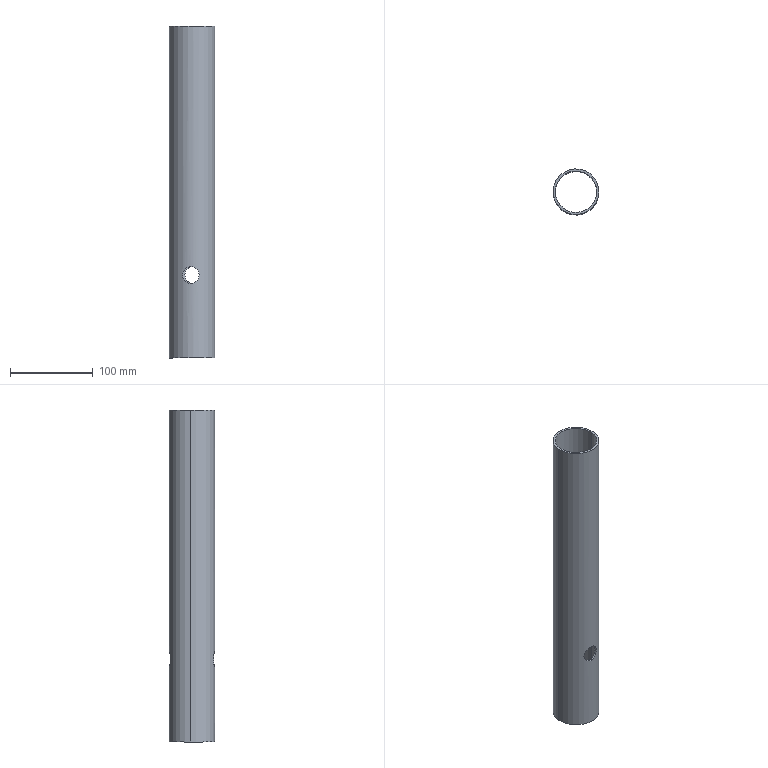Component | SolidWorks | 7LegTravel-2 | 1 solid | 10 faces | box 55 x 55 x 400 mm | volume 163332 mm3 | cylinder 8 | plane 2 | commonest cylinder face diameters 20 x4 50 x2 55 x2
build123d program:
from build123d import *

# Parameters (mm, degrees)
SKETCH1_R           = 27.5
SKETCH1_R_2         = 25
BOSS_EXTRUDE1_DEPTH = 400
SKETCH2_R           = 10
CUT_EXTRUDE1_DEPTH  = 240


with BuildPart() as part:
    # Sketch1 → Boss-Extrude1 (new body)
    with BuildSketch(Plane.XY):
        Circle(SKETCH1_R)
        Circle(SKETCH1_R_2, mode=Mode.SUBTRACT)
    extrude(amount=BOSS_EXTRUDE1_DEPTH)

    # Sketch2 → Cut-Extrude1 (cut, symmetric)
    with BuildSketch(Plane(origin=(0, 25, 0), x_dir=(1, 0, 0), z_dir=(0, 1, 0))):
        with Locations(Location((0, -300, 0), (0, 0, 270))):
            Circle(SKETCH2_R)
    extrude(amount=CUT_EXTRUDE1_DEPTH, both=True, mode=Mode.SUBTRACT)


solid = part.part

# Placed as in the assembly
solid = solid.moved(Location((142.5, 813.71, 917.68), (-180, 0, -176.706)))
STEP:
#1=CARTESIAN_POINT('',(5.548,30.955,24.712));
#2=VERTEX_POINT('',#1);
#3=CARTESIAN_POINT('',(5.548,30.955,23.924));
#4=VERTEX_POINT('',#3);
#5=CARTESIAN_POINT('',(5.548,30.955,24.712));
#6=CARTESIAN_POINT('',(5.561,30.954,24.712));
#7=CARTESIAN_POINT('',(5.574,30.954,24.711));
#8=CARTESIAN_POINT('',(5.6,30.953,24.709));
#9=CARTESIAN_POINT('',(5.613,30.953,24.707));
#10=CARTESIAN_POINT('',(5.651,30.954,24.699));
#11=CARTESIAN_POINT('',(5.676,30.955,24.691));
#12=CARTESIAN_POINT('',(5.712,30.958,24.677));
#13=CARTESIAN_POINT('',(5.724,30.959,24.671));
#14=CARTESIAN_POINT('',(5.747,30.962,24.659));
#15=CARTESIAN_POINT('',(5.758,30.963,24.652));
#16=CARTESIAN_POINT('',(5.79,30.968,24.631));
#17=CARTESIAN_POINT('',(5.81,30.972,24.615));
#18=CARTESIAN_POINT('',(5.847,30.979,24.578));
#19=CARTESIAN_POINT('',(5.863,30.983,24.558));
#20=CARTESIAN_POINT('',(5.885,30.988,24.527));
#21=CARTESIAN_POINT('',(5.891,30.99,24.516));
#22=CARTESIAN_POINT('',(5.904,30.994,24.493));
#23=CARTESIAN_POINT('',(5.91,30.995,24.481));
#24=CARTESIAN_POINT('',(5.925,31.,24.445));
#25=CARTESIAN_POINT('',(5.932,31.002,24.421));
#26=CARTESIAN_POINT('',(5.94,31.005,24.383));
#27=CARTESIAN_POINT('',(5.942,31.005,24.37));
#28=CARTESIAN_POINT('',(5.945,31.006,24.344));
#29=CARTESIAN_POINT('',(5.945,31.006,24.331));
#30=CARTESIAN_POINT('',(5.945,31.006,24.292));
#31=CARTESIAN_POINT('',(5.943,31.005,24.266));
#32=CARTESIAN_POINT('',(5.935,31.003,24.228));
#33=CARTESIAN_POINT('',(5.932,31.002,24.215));
#34=CARTESIAN_POINT('',(5.924,31.,24.191));
#35=CARTESIAN_POINT('',(5.919,30.998,24.178));
#36=CARTESIAN_POINT('',(5.909,30.995,24.155));
#37=CARTESIAN_POINT('',(5.904,30.994,24.143));
#38=CARTESIAN_POINT('',(5.891,30.99,24.12));
#39=CARTESIAN_POINT('',(5.885,30.988,24.109));
#40=CARTESIAN_POINT('',(5.863,30.983,24.077));
#41=CARTESIAN_POINT('',(5.846,30.979,24.058));
#42=CARTESIAN_POINT('',(5.81,30.972,24.022));
#43=CARTESIAN_POINT('',(5.789,30.968,24.005));
#44=CARTESIAN_POINT('',(5.747,30.962,23.977));
#45=CARTESIAN_POINT('',(5.724,30.959,23.965));
#46=CARTESIAN_POINT('',(5.688,30.956,23.95));
#47=CARTESIAN_POINT('',(5.675,30.955,23.945));
#48=CARTESIAN_POINT('',(5.651,30.954,23.938));
#49=CARTESIAN_POINT('',(5.638,30.953,23.935));
#50=CARTESIAN_POINT('',(5.6,30.953,23.927));
#51=CARTESIAN_POINT('',(5.574,30.953,23.924));
#52=CARTESIAN_POINT('',(5.548,30.955,23.924));
#53=B_SPLINE_CURVE_WITH_KNOTS('',3,(#5,#6,#7,#8,#9,#10,#11,#12,#13,#14,#15,#16,#17,#18,#19,#20,#21,#22,#23,#24,#25,#26,#27,#28,#29,#30,#31,#32,#33,#34,#35,#36,#37,#38,#39,#40,#41,#42,#43,#44,#45,#46,#47,#48,#49,#50,#51,#52),.UNSPECIFIED.,.F.,.F.,(4,2,2,2,2,2,2,2,2,2,2,2,2,2,2,2,2,2,2,2,2,2,2,4),(0.03154,0.03252,0.03351,0.03548,0.03646,0.03745,0.03942,0.04139,0.04238,0.04336,0.04533,0.04632,0.0473,0.04927,0.05026,0.05124,0.05223,0.05321,0.05519,0.05716,0.05913,0.06011,0.0611,0.06307),.UNSPECIFIED.);
#54=EDGE_CURVE('',#2,#4,#53,.T.);
#55=ORIENTED_EDGE('',*,*,#54,.F.);
#56=CARTESIAN_POINT('',(5.554,31.053,24.712));
#57=VERTEX_POINT('',#56);
#58=CARTESIAN_POINT('',(5.124,23.585,24.712));
#59=DIRECTION('',(0.05742,0.9983,0.));
#60=VECTOR('',#59,39.37);
#61=LINE('',#58,#60);
#62=EDGE_CURVE('',#2,#57,#61,.T.);
#63=ORIENTED_EDGE('',*,*,#62,.T.);
#64=CARTESIAN_POINT('',(5.554,31.053,23.924));
#65=VERTEX_POINT('',#64);
#66=CARTESIAN_POINT('',(5.554,31.053,24.712));
#67=CARTESIAN_POINT('',(5.567,31.052,24.712));
#68=CARTESIAN_POINT('',(5.58,31.052,24.711));
#69=CARTESIAN_POINT('',(5.606,31.051,24.709));
#70=CARTESIAN_POINT('',(5.619,31.052,24.707));
#71=CARTESIAN_POINT('',(5.657,31.052,24.699));
#72=CARTESIAN_POINT('',(5.682,31.054,24.691));
#73=CARTESIAN_POINT('',(5.718,31.057,24.676));
#74=CARTESIAN_POINT('',(5.73,31.059,24.671));
#75=CARTESIAN_POINT('',(5.753,31.062,24.659));
#76=CARTESIAN_POINT('',(5.764,31.064,24.652));
#77=CARTESIAN_POINT('',(5.796,31.069,24.631));
#78=CARTESIAN_POINT('',(5.816,31.073,24.614));
#79=CARTESIAN_POINT('',(5.853,31.082,24.578));
#80=CARTESIAN_POINT('',(5.869,31.086,24.558));
#81=CARTESIAN_POINT('',(5.891,31.092,24.527));
#82=CARTESIAN_POINT('',(5.897,31.094,24.516));
#83=CARTESIAN_POINT('',(5.91,31.098,24.493));
#84=CARTESIAN_POINT('',(5.915,31.1,24.481));
#85=CARTESIAN_POINT('',(5.931,31.105,24.446));
#86=CARTESIAN_POINT('',(5.938,31.108,24.421));
#87=CARTESIAN_POINT('',(5.946,31.111,24.383));
#88=CARTESIAN_POINT('',(5.948,31.111,24.37));
#89=CARTESIAN_POINT('',(5.951,31.112,24.344));
#90=CARTESIAN_POINT('',(5.951,31.113,24.331));
#91=CARTESIAN_POINT('',(5.951,31.113,24.292));
#92=CARTESIAN_POINT('',(5.949,31.112,24.266));
#93=CARTESIAN_POINT('',(5.941,31.109,24.228));
#94=CARTESIAN_POINT('',(5.938,31.108,24.215));
#95=CARTESIAN_POINT('',(5.93,31.105,24.191));
#96=CARTESIAN_POINT('',(5.926,31.103,24.178));
#97=CARTESIAN_POINT('',(5.915,31.1,24.155));
#98=CARTESIAN_POINT('',(5.91,31.098,24.143));
#99=CARTESIAN_POINT('',(5.897,31.094,24.12));
#100=CARTESIAN_POINT('',(5.891,31.092,24.109));
#101=CARTESIAN_POINT('',(5.869,31.086,24.078));
#102=CARTESIAN_POINT('',(5.852,31.082,24.058));
#103=CARTESIAN_POINT('',(5.825,31.075,24.031));
#104=CARTESIAN_POINT('',(5.815,31.073,24.022));
#105=CARTESIAN_POINT('',(5.795,31.069,24.006));
#106=CARTESIAN_POINT('',(5.785,31.067,23.998));
#107=CARTESIAN_POINT('',(5.753,31.062,23.977));
#108=CARTESIAN_POINT('',(5.73,31.059,23.965));
#109=CARTESIAN_POINT('',(5.694,31.055,23.95));
#110=CARTESIAN_POINT('',(5.681,31.054,23.945));
#111=CARTESIAN_POINT('',(5.657,31.053,23.938));
#112=CARTESIAN_POINT('',(5.644,31.052,23.935));
#113=CARTESIAN_POINT('',(5.619,31.052,23.93));
#114=CARTESIAN_POINT('',(5.606,31.051,23.928));
#115=CARTESIAN_POINT('',(5.58,31.052,23.925));
#116=CARTESIAN_POINT('',(5.567,31.052,23.924));
#117=CARTESIAN_POINT('',(5.554,31.053,23.924));
#118=B_SPLINE_CURVE_WITH_KNOTS('',3,(#66,#67,#68,#69,#70,#71,#72,#73,#74,#75,#76,#77,#78,#79,#80,#81,#82,#83,#84,#85,#86,#87,#88,#89,#90,#91,#92,#93,#94,#95,#96,#97,#98,#99,#100,#101,#102,#103,#104,#105,#106,#107,#108,#109,#110,#111,#112,#113,#114,#115,#116,#117),.UNSPECIFIED.,.F.,.F.,(4,2,2,2,2,2,2,2,2,2,2,2,2,2,2,2,2,2,2,2,2,2,2,2,2,4),(0.0316,0.03259,0.03357,0.03555,0.03653,0.03752,0.03949,0.04147,0.04245,0.04344,0.04541,0.0464,0.04739,0.04936,0.05035,0.05134,0.05232,0.05331,0.05528,0.05627,0.05726,0.05923,0.06022,0.0612,0.06219,0.06318),.UNSPECIFIED.);
#119=EDGE_CURVE('',#57,#65,#118,.T.);
#120=ORIENTED_EDGE('',*,*,#119,.T.);
#121=CARTESIAN_POINT('',(5.124,23.585,23.924));
#122=DIRECTION('',(0.05742,0.9983,0.));
#123=VECTOR('',#122,39.37);
#124=LINE('',#121,#123);
#125=EDGE_CURVE('',#4,#65,#124,.T.);
#126=ORIENTED_EDGE('',*,*,#125,.F.);
#127=EDGE_LOOP('',(#55,#63,#120,#126));
#128=FACE_OUTER_BOUND('',#127,.T.);
#129=CARTESIAN_POINT('',(5.124,23.585,24.318));
#130=DIRECTION('',(0.05742,0.9983,0.));
#131=DIRECTION('',(0.,0.,-1.));
#132=AXIS2_PLACEMENT_3D('',#129,#130,#131);
#133=CYLINDRICAL_SURFACE('',#132,0.3937);
#134=ADVANCED_FACE('',(#128),#133,.F.);
#135=CARTESIAN_POINT('',(5.667,33.018,23.924));
#136=VERTEX_POINT('',#135);
#137=CARTESIAN_POINT('',(5.667,33.018,24.712));
#138=VERTEX_POINT('',#137);
#139=CARTESIAN_POINT('',(5.667,33.018,23.924));
#140=CARTESIAN_POINT('',(5.693,33.017,23.924));
#141=CARTESIAN_POINT('',(5.719,33.014,23.927));
#142=CARTESIAN_POINT('',(5.757,33.009,23.935));
#143=CARTESIAN_POINT('',(5.769,33.007,23.938));
#144=CARTESIAN_POINT('',(5.794,33.003,23.945));
#145=CARTESIAN_POINT('',(5.806,33.001,23.95));
#146=CARTESIAN_POINT('',(5.841,32.993,23.965));
#147=CARTESIAN_POINT('',(5.863,32.987,23.977));
#148=CARTESIAN_POINT('',(5.895,32.978,23.998));
#149=CARTESIAN_POINT('',(5.905,32.975,24.006));
#150=CARTESIAN_POINT('',(5.924,32.969,24.022));
#151=CARTESIAN_POINT('',(5.934,32.965,24.031));
#152=CARTESIAN_POINT('',(5.96,32.956,24.058));
#153=CARTESIAN_POINT('',(5.976,32.95,24.078));
#154=CARTESIAN_POINT('',(6.004,32.938,24.12));
#155=CARTESIAN_POINT('',(6.016,32.933,24.143));
#156=CARTESIAN_POINT('',(6.03,32.926,24.178));
#157=CARTESIAN_POINT('',(6.035,32.924,24.19));
#158=CARTESIAN_POINT('',(6.042,32.92,24.215));
#159=CARTESIAN_POINT('',(6.045,32.919,24.228));
#160=CARTESIAN_POINT('',(6.053,32.915,24.266));
#161=CARTESIAN_POINT('',(6.055,32.914,24.292));
#162=CARTESIAN_POINT('',(6.055,32.914,24.331));
#163=CARTESIAN_POINT('',(6.054,32.914,24.344));
#164=CARTESIAN_POINT('',(6.052,32.915,24.37));
#165=CARTESIAN_POINT('',(6.05,32.916,24.383));
#166=CARTESIAN_POINT('',(6.043,32.92,24.421));
#167=CARTESIAN_POINT('',(6.035,32.924,24.446));
#168=CARTESIAN_POINT('',(6.016,32.933,24.494));
#169=CARTESIAN_POINT('',(6.004,32.938,24.516));
#170=CARTESIAN_POINT('',(5.983,32.947,24.548));
#171=CARTESIAN_POINT('',(5.976,32.95,24.558));
#172=CARTESIAN_POINT('',(5.96,32.956,24.578));
#173=CARTESIAN_POINT('',(5.951,32.959,24.588));
#174=CARTESIAN_POINT('',(5.925,32.969,24.615));
#175=CARTESIAN_POINT('',(5.905,32.975,24.631));
#176=CARTESIAN_POINT('',(5.874,32.984,24.652));
#177=CARTESIAN_POINT('',(5.863,32.987,24.659));
#178=CARTESIAN_POINT('',(5.84,32.993,24.671));
#179=CARTESIAN_POINT('',(5.829,32.996,24.677));
#180=CARTESIAN_POINT('',(5.794,33.003,24.691));
#181=CARTESIAN_POINT('',(5.769,33.007,24.699));
#182=CARTESIAN_POINT('',(5.731,33.013,24.707));
#183=CARTESIAN_POINT('',(5.718,33.014,24.709));
#184=CARTESIAN_POINT('',(5.693,33.017,24.711));
#185=CARTESIAN_POINT('',(5.68,33.018,24.712));
#186=CARTESIAN_POINT('',(5.667,33.018,24.712));
#187=B_SPLINE_CURVE_WITH_KNOTS('',3,(#139,#140,#141,#142,#143,#144,#145,#146,#147,#148,#149,#150,#151,#152,#153,#154,#155,#156,#157,#158,#159,#160,#161,#162,#163,#164,#165,#166,#167,#168,#169,#170,#171,#172,#173,#174,#175,#176,#177,#178,#179,#180,#181,#182,#183,#184,#185,#186),.UNSPECIFIED.,.F.,.F.,(4,2,2,2,2,2,2,2,2,2,2,2,2,2,2,2,2,2,2,2,2,2,2,4),(0.,0.001975,0.002962,0.00395,0.005925,0.006912,0.0079,0.009875,0.01185,0.01284,0.01382,0.0158,0.01679,0.01777,0.01975,0.02172,0.02271,0.0237,0.02567,0.02666,0.02765,0.02962,0.03061,0.0316),.UNSPECIFIED.);
#188=EDGE_CURVE('',#136,#138,#187,.T.);
#189=ORIENTED_EDGE('',*,*,#188,.T.);
#190=CARTESIAN_POINT('',(5.672,33.117,24.712));
#191=VERTEX_POINT('',#190);
#192=CARTESIAN_POINT('',(5.124,23.585,24.712));
#193=DIRECTION('',(0.05742,0.9983,0.));
#194=VECTOR('',#193,39.37);
#195=LINE('',#192,#194);
#196=EDGE_CURVE('',#138,#191,#195,.T.);
#197=ORIENTED_EDGE('',*,*,#196,.T.);
#198=CARTESIAN_POINT('',(5.672,33.117,23.924));
#199=VERTEX_POINT('',#198);
#200=CARTESIAN_POINT('',(5.672,33.117,23.924));
#201=CARTESIAN_POINT('',(5.699,33.115,23.924));
#202=CARTESIAN_POINT('',(5.724,33.113,23.927));
#203=CARTESIAN_POINT('',(5.762,33.108,23.935));
#204=CARTESIAN_POINT('',(5.774,33.106,23.938));
#205=CARTESIAN_POINT('',(5.799,33.102,23.945));
#206=CARTESIAN_POINT('',(5.811,33.1,23.95));
#207=CARTESIAN_POINT('',(5.847,33.093,23.965));
#208=CARTESIAN_POINT('',(5.869,33.087,23.977));
#209=CARTESIAN_POINT('',(5.9,33.079,23.998));
#210=CARTESIAN_POINT('',(5.911,33.076,24.006));
#211=CARTESIAN_POINT('',(5.93,33.07,24.022));
#212=CARTESIAN_POINT('',(5.94,33.067,24.031));
#213=CARTESIAN_POINT('',(5.966,33.059,24.058));
#214=CARTESIAN_POINT('',(5.982,33.053,24.078));
#215=CARTESIAN_POINT('',(6.01,33.042,24.12));
#216=CARTESIAN_POINT('',(6.022,33.037,24.143));
#217=CARTESIAN_POINT('',(6.036,33.031,24.178));
#218=CARTESIAN_POINT('',(6.041,33.029,24.191));
#219=CARTESIAN_POINT('',(6.048,33.026,24.215));
#220=CARTESIAN_POINT('',(6.051,33.025,24.228));
#221=CARTESIAN_POINT('',(6.059,33.021,24.266));
#222=CARTESIAN_POINT('',(6.061,33.02,24.292));
#223=CARTESIAN_POINT('',(6.061,33.02,24.331));
#224=CARTESIAN_POINT('',(6.061,33.02,24.344));
#225=CARTESIAN_POINT('',(6.058,33.022,24.37));
#226=CARTESIAN_POINT('',(6.056,33.022,24.383));
#227=CARTESIAN_POINT('',(6.049,33.026,24.421));
#228=CARTESIAN_POINT('',(6.041,33.029,24.446));
#229=CARTESIAN_POINT('',(6.022,33.037,24.493));
#230=CARTESIAN_POINT('',(6.01,33.042,24.516));
#231=CARTESIAN_POINT('',(5.989,33.05,24.548));
#232=CARTESIAN_POINT('',(5.982,33.053,24.558));
#233=CARTESIAN_POINT('',(5.966,33.059,24.578));
#234=CARTESIAN_POINT('',(5.957,33.061,24.588));
#235=CARTESIAN_POINT('',(5.93,33.07,24.615));
#236=CARTESIAN_POINT('',(5.911,33.076,24.631));
#237=CARTESIAN_POINT('',(5.88,33.085,24.652));
#238=CARTESIAN_POINT('',(5.869,33.087,24.659));
#239=CARTESIAN_POINT('',(5.846,33.093,24.671));
#240=CARTESIAN_POINT('',(5.835,33.095,24.677));
#241=CARTESIAN_POINT('',(5.799,33.102,24.691));
#242=CARTESIAN_POINT('',(5.775,33.106,24.699));
#243=CARTESIAN_POINT('',(5.737,33.111,24.707));
#244=CARTESIAN_POINT('',(5.724,33.113,24.709));
#245=CARTESIAN_POINT('',(5.698,33.115,24.711));
#246=CARTESIAN_POINT('',(5.685,33.116,24.712));
#247=CARTESIAN_POINT('',(5.672,33.117,24.712));
#248=B_SPLINE_CURVE_WITH_KNOTS('',3,(#200,#201,#202,#203,#204,#205,#206,#207,#208,#209,#210,#211,#212,#213,#214,#215,#216,#217,#218,#219,#220,#221,#222,#223,#224,#225,#226,#227,#228,#229,#230,#231,#232,#233,#234,#235,#236,#237,#238,#239,#240,#241,#242,#243,#244,#245,#246,#247),.UNSPECIFIED.,.F.,.F.,(4,2,2,2,2,2,2,2,2,2,2,2,2,2,2,2,2,2,2,2,2,2,2,4),(0.,0.001971,0.002957,0.003942,0.005913,0.006899,0.007884,0.009855,0.01183,0.01281,0.0138,0.01577,0.01675,0.01774,0.01971,0.02168,0.02267,0.02365,0.02562,0.02661,0.0276,0.02957,0.03055,0.03154),.UNSPECIFIED.);
#249=EDGE_CURVE('',#199,#191,#248,.T.);
#250=ORIENTED_EDGE('',*,*,#249,.F.);
#251=CARTESIAN_POINT('',(5.124,23.585,23.924));
#252=DIRECTION('',(0.05742,0.9983,0.));
#253=VECTOR('',#252,39.37);
#254=LINE('',#251,#253);
#255=EDGE_CURVE('',#136,#199,#254,.T.);
#256=ORIENTED_EDGE('',*,*,#255,.F.);
#257=EDGE_LOOP('',(#189,#197,#250,#256));
#258=FACE_OUTER_BOUND('',#257,.T.);
#259=CARTESIAN_POINT('',(5.124,23.585,24.318));
#260=DIRECTION('',(0.05742,0.9983,0.));
#261=DIRECTION('',(0.,0.,-1.));
#262=AXIS2_PLACEMENT_3D('',#259,#260,#261);
#263=CYLINDRICAL_SURFACE('',#262,0.3937);
#264=ADVANCED_FACE('',(#258),#263,.F.);
#265=CARTESIAN_POINT('',(5.554,31.053,23.924));
#266=CARTESIAN_POINT('',(5.527,31.055,23.924));
#267=CARTESIAN_POINT('',(5.502,31.057,23.927));
#268=CARTESIAN_POINT('',(5.464,31.062,23.935));
#269=CARTESIAN_POINT('',(5.451,31.064,23.938));
#270=CARTESIAN_POINT('',(5.427,31.069,23.945));
#271=CARTESIAN_POINT('',(5.415,31.071,23.95));
#272=CARTESIAN_POINT('',(5.379,31.079,23.965));
#273=CARTESIAN_POINT('',(5.357,31.084,23.977));
#274=CARTESIAN_POINT('',(5.326,31.094,23.998));
#275=CARTESIAN_POINT('',(5.315,31.097,24.006));
#276=CARTESIAN_POINT('',(5.296,31.103,24.022));
#277=CARTESIAN_POINT('',(5.287,31.106,24.031));
#278=CARTESIAN_POINT('',(5.26,31.116,24.058));
#279=CARTESIAN_POINT('',(5.244,31.122,24.078));
#280=CARTESIAN_POINT('',(5.216,31.134,24.12));
#281=CARTESIAN_POINT('',(5.205,31.139,24.143));
#282=CARTESIAN_POINT('',(5.19,31.146,24.178));
#283=CARTESIAN_POINT('',(5.186,31.148,24.19));
#284=CARTESIAN_POINT('',(5.178,31.151,24.215));
#285=CARTESIAN_POINT('',(5.175,31.153,24.228));
#286=CARTESIAN_POINT('',(5.168,31.157,24.266));
#287=CARTESIAN_POINT('',(5.165,31.158,24.292));
#288=CARTESIAN_POINT('',(5.165,31.158,24.331));
#289=CARTESIAN_POINT('',(5.166,31.158,24.344));
#290=CARTESIAN_POINT('',(5.169,31.156,24.37));
#291=CARTESIAN_POINT('',(5.17,31.155,24.383));
#292=CARTESIAN_POINT('',(5.178,31.152,24.421));
#293=CARTESIAN_POINT('',(5.185,31.148,24.446));
#294=CARTESIAN_POINT('',(5.205,31.139,24.494));
#295=CARTESIAN_POINT('',(5.217,31.134,24.516));
#296=CARTESIAN_POINT('',(5.237,31.125,24.548));
#297=CARTESIAN_POINT('',(5.245,31.122,24.558));
#298=CARTESIAN_POINT('',(5.261,31.116,24.578));
#299=CARTESIAN_POINT('',(5.269,31.112,24.588));
#300=CARTESIAN_POINT('',(5.296,31.103,24.615));
#301=CARTESIAN_POINT('',(5.315,31.097,24.631));
#302=CARTESIAN_POINT('',(5.347,31.087,24.652));
#303=CARTESIAN_POINT('',(5.358,31.084,24.659));
#304=CARTESIAN_POINT('',(5.38,31.079,24.671));
#305=CARTESIAN_POINT('',(5.391,31.076,24.677));
#306=CARTESIAN_POINT('',(5.427,31.069,24.691));
#307=CARTESIAN_POINT('',(5.451,31.064,24.699));
#308=CARTESIAN_POINT('',(5.489,31.059,24.707));
#309=CARTESIAN_POINT('',(5.502,31.057,24.709));
#310=CARTESIAN_POINT('',(5.528,31.055,24.711));
#311=CARTESIAN_POINT('',(5.541,31.054,24.712));
#312=CARTESIAN_POINT('',(5.554,31.053,24.712));
#313=B_SPLINE_CURVE_WITH_KNOTS('',3,(#265,#266,#267,#268,#269,#270,#271,#272,#273,#274,#275,#276,#277,#278,#279,#280,#281,#282,#283,#284,#285,#286,#287,#288,#289,#290,#291,#292,#293,#294,#295,#296,#297,#298,#299,#300,#301,#302,#303,#304,#305,#306,#307,#308,#309,#310,#311,#312),.UNSPECIFIED.,.F.,.F.,(4,2,2,2,2,2,2,2,2,2,2,2,2,2,2,2,2,2,2,2,2,2,2,4),(0.,0.001975,0.002962,0.00395,0.005925,0.006912,0.0079,0.009875,0.01185,0.01284,0.01382,0.0158,0.01679,0.01777,0.01975,0.02172,0.02271,0.0237,0.02567,0.02666,0.02765,0.02962,0.03061,0.0316),.UNSPECIFIED.);
#314=EDGE_CURVE('',#65,#57,#313,.T.);
#315=ORIENTED_EDGE('',*,*,#314,.F.);
#316=ORIENTED_EDGE('',*,*,#119,.F.);
#317=EDGE_LOOP('',(#315,#316));
#318=FACE_BOUND('',#317,.T.);
#319=CARTESIAN_POINT('',(6.593,31.979,20.381));
#320=VERTEX_POINT('',#319);
#321=CARTESIAN_POINT('',(4.628,32.092,20.381));
#322=VERTEX_POINT('',#321);
#323=CARTESIAN_POINT('',(5.61,32.036,20.381));
#324=DIRECTION('',(0.,0.,-1.));
#325=DIRECTION('',(-0.9983,0.05742,-0.));
#326=AXIS2_PLACEMENT_3D('',#323,#324,#325);
#327=CIRCLE('',#326,0.9843);
#328=EDGE_CURVE('',#320,#322,#327,.T.);
#329=ORIENTED_EDGE('',*,*,#328,.T.);
#330=CARTESIAN_POINT('',(4.628,32.092,36.129));
#331=VERTEX_POINT('',#330);
#332=CARTESIAN_POINT('',(4.628,32.092,20.381));
#333=DIRECTION('',(-0.,-0.,1.));
#334=VECTOR('',#333,39.37);
#335=LINE('',#332,#334);
#336=EDGE_CURVE('',#322,#331,#335,.T.);
#337=ORIENTED_EDGE('',*,*,#336,.T.);
#338=CARTESIAN_POINT('',(6.593,31.979,36.129));
#339=VERTEX_POINT('',#338);
#340=CARTESIAN_POINT('',(5.61,32.036,36.129));
#341=DIRECTION('',(0.,0.,-1.));
#342=DIRECTION('',(-0.9983,0.05742,-0.));
#343=AXIS2_PLACEMENT_3D('',#340,#341,#342);
#344=CIRCLE('',#343,0.9843);
#345=EDGE_CURVE('',#339,#331,#344,.T.);
#346=ORIENTED_EDGE('',*,*,#345,.F.);
#347=CARTESIAN_POINT('',(6.593,31.979,20.381));
#348=DIRECTION('',(-0.,-0.,1.));
#349=VECTOR('',#348,39.37);
#350=LINE('',#347,#349);
#351=EDGE_CURVE('',#320,#339,#350,.T.);
#352=ORIENTED_EDGE('',*,*,#351,.F.);
#353=EDGE_LOOP('',(#329,#337,#346,#352));
#354=FACE_OUTER_BOUND('',#353,.T.);
#355=CARTESIAN_POINT('',(5.61,32.036,20.381));
#356=DIRECTION('',(-0.,-0.,1.));
#357=DIRECTION('',(0.9983,-0.05742,0.));
#358=AXIS2_PLACEMENT_3D('',#355,#356,#357);
#359=CYLINDRICAL_SURFACE('',#358,0.9843);
#360=ADVANCED_FACE('',(#318,#354),#359,.F.);
#361=ORIENTED_EDGE('',*,*,#249,.T.);
#362=CARTESIAN_POINT('',(5.672,33.117,24.712));
#363=CARTESIAN_POINT('',(5.659,33.117,24.712));
#364=CARTESIAN_POINT('',(5.647,33.118,24.711));
#365=CARTESIAN_POINT('',(5.621,33.119,24.709));
#366=CARTESIAN_POINT('',(5.608,33.119,24.707));
#367=CARTESIAN_POINT('',(5.569,33.118,24.699));
#368=CARTESIAN_POINT('',(5.545,33.117,24.691));
#369=CARTESIAN_POINT('',(5.509,33.114,24.677));
#370=CARTESIAN_POINT('',(5.497,33.113,24.671));
#371=CARTESIAN_POINT('',(5.474,33.11,24.659));
#372=CARTESIAN_POINT('',(5.463,33.108,24.652));
#373=CARTESIAN_POINT('',(5.431,33.104,24.631));
#374=CARTESIAN_POINT('',(5.411,33.1,24.615));
#375=CARTESIAN_POINT('',(5.374,33.093,24.578));
#376=CARTESIAN_POINT('',(5.357,33.089,24.558));
#377=CARTESIAN_POINT('',(5.336,33.083,24.527));
#378=CARTESIAN_POINT('',(5.329,33.081,24.516));
#379=CARTESIAN_POINT('',(5.317,33.078,24.493));
#380=CARTESIAN_POINT('',(5.311,33.076,24.481));
#381=CARTESIAN_POINT('',(5.296,33.072,24.445));
#382=CARTESIAN_POINT('',(5.288,33.069,24.421));
#383=CARTESIAN_POINT('',(5.28,33.067,24.383));
#384=CARTESIAN_POINT('',(5.278,33.066,24.37));
#385=CARTESIAN_POINT('',(5.276,33.066,24.344));
#386=CARTESIAN_POINT('',(5.275,33.065,24.331));
#387=CARTESIAN_POINT('',(5.275,33.065,24.292));
#388=CARTESIAN_POINT('',(5.278,33.066,24.266));
#389=CARTESIAN_POINT('',(5.286,33.069,24.228));
#390=CARTESIAN_POINT('',(5.289,33.07,24.215));
#391=CARTESIAN_POINT('',(5.297,33.072,24.191));
#392=CARTESIAN_POINT('',(5.301,33.073,24.178));
#393=CARTESIAN_POINT('',(5.311,33.076,24.155));
#394=CARTESIAN_POINT('',(5.317,33.078,24.143));
#395=CARTESIAN_POINT('',(5.329,33.081,24.12));
#396=CARTESIAN_POINT('',(5.336,33.083,24.109));
#397=CARTESIAN_POINT('',(5.358,33.089,24.077));
#398=CARTESIAN_POINT('',(5.374,33.093,24.058));
#399=CARTESIAN_POINT('',(5.411,33.1,24.022));
#400=CARTESIAN_POINT('',(5.431,33.104,24.005));
#401=CARTESIAN_POINT('',(5.474,33.11,23.977));
#402=CARTESIAN_POINT('',(5.497,33.113,23.965));
#403=CARTESIAN_POINT('',(5.533,33.116,23.95));
#404=CARTESIAN_POINT('',(5.545,33.117,23.945));
#405=CARTESIAN_POINT('',(5.57,33.118,23.938));
#406=CARTESIAN_POINT('',(5.582,33.118,23.935));
#407=CARTESIAN_POINT('',(5.62,33.119,23.927));
#408=CARTESIAN_POINT('',(5.646,33.118,23.924));
#409=CARTESIAN_POINT('',(5.672,33.117,23.924));
#410=B_SPLINE_CURVE_WITH_KNOTS('',3,(#362,#363,#364,#365,#366,#367,#368,#369,#370,#371,#372,#373,#374,#375,#376,#377,#378,#379,#380,#381,#382,#383,#384,#385,#386,#387,#388,#389,#390,#391,#392,#393,#394,#395,#396,#397,#398,#399,#400,#401,#402,#403,#404,#405,#406,#407,#408,#409),.UNSPECIFIED.,.F.,.F.,(4,2,2,2,2,2,2,2,2,2,2,2,2,2,2,2,2,2,2,2,2,2,2,4),(0.03154,0.03252,0.03351,0.03548,0.03646,0.03745,0.03942,0.04139,0.04238,0.04336,0.04533,0.04632,0.0473,0.04927,0.05026,0.05124,0.05223,0.05321,0.05519,0.05716,0.05913,0.06011,0.0611,0.06307),.UNSPECIFIED.);
#411=EDGE_CURVE('',#191,#199,#410,.T.);
#412=ORIENTED_EDGE('',*,*,#411,.T.);
#413=EDGE_LOOP('',(#361,#412));
#414=FACE_BOUND('',#413,.T.);
#415=CARTESIAN_POINT('',(4.529,32.098,20.381));
#416=VERTEX_POINT('',#415);
#417=CARTESIAN_POINT('',(6.691,31.974,20.381));
#418=VERTEX_POINT('',#417);
#419=CARTESIAN_POINT('',(5.61,32.036,20.381));
#420=DIRECTION('',(0.,0.,-1.));
#421=DIRECTION('',(-0.9983,0.05742,-0.));
#422=AXIS2_PLACEMENT_3D('',#419,#420,#421);
#423=CIRCLE('',#422,1.083);
#424=EDGE_CURVE('',#416,#418,#423,.T.);
#425=ORIENTED_EDGE('',*,*,#424,.F.);
#426=CARTESIAN_POINT('',(4.529,32.098,36.129));
#427=VERTEX_POINT('',#426);
#428=CARTESIAN_POINT('',(4.529,32.098,20.381));
#429=DIRECTION('',(-0.,-0.,1.));
#430=VECTOR('',#429,39.37);
#431=LINE('',#428,#430);
#432=EDGE_CURVE('',#416,#427,#431,.T.);
#433=ORIENTED_EDGE('',*,*,#432,.T.);
#434=CARTESIAN_POINT('',(6.691,31.974,36.129));
#435=VERTEX_POINT('',#434);
#436=CARTESIAN_POINT('',(5.61,32.036,36.129));
#437=DIRECTION('',(0.,0.,-1.));
#438=DIRECTION('',(-0.9983,0.05742,-0.));
#439=AXIS2_PLACEMENT_3D('',#436,#437,#438);
#440=CIRCLE('',#439,1.083);
#441=EDGE_CURVE('',#427,#435,#440,.T.);
#442=ORIENTED_EDGE('',*,*,#441,.T.);
#443=CARTESIAN_POINT('',(6.691,31.974,20.381));
#444=DIRECTION('',(-0.,-0.,1.));
#445=VECTOR('',#444,39.37);
#446=LINE('',#443,#445);
#447=EDGE_CURVE('',#418,#435,#446,.T.);
#448=ORIENTED_EDGE('',*,*,#447,.F.);
#449=EDGE_LOOP('',(#425,#433,#442,#448));
#450=FACE_OUTER_BOUND('',#449,.T.);
#451=CARTESIAN_POINT('',(5.61,32.036,20.381));
#452=DIRECTION('',(-0.,-0.,1.));
#453=DIRECTION('',(0.9983,-0.05742,0.));
#454=AXIS2_PLACEMENT_3D('',#451,#452,#453);
#455=CYLINDRICAL_SURFACE('',#454,1.083);
#456=ADVANCED_FACE('',(#414,#450),#455,.T.);
#457=CARTESIAN_POINT('',(5.61,32.036,20.381));
#458=DIRECTION('',(0.,0.,-1.));
#459=DIRECTION('',(-0.9983,0.05742,-0.));
#460=AXIS2_PLACEMENT_3D('',#457,#458,#459);
#461=CIRCLE('',#460,1.083);
#462=EDGE_CURVE('',#418,#416,#461,.T.);
#463=ORIENTED_EDGE('',*,*,#462,.T.);
#464=ORIENTED_EDGE('',*,*,#424,.T.);
#465=EDGE_LOOP('',(#463,#464));
#466=FACE_OUTER_BOUND('',#465,.T.);
#467=ORIENTED_EDGE('',*,*,#328,.F.);
#468=CARTESIAN_POINT('',(5.61,32.036,20.381));
#469=DIRECTION('',(0.,0.,-1.));
#470=DIRECTION('',(-0.9983,0.05742,-0.));
#471=AXIS2_PLACEMENT_3D('',#468,#469,#470);
#472=CIRCLE('',#471,0.9843);
#473=EDGE_CURVE('',#322,#320,#472,.T.);
#474=ORIENTED_EDGE('',*,*,#473,.F.);
#475=EDGE_LOOP('',(#467,#474));
#476=FACE_BOUND('',#475,.T.);
#477=CARTESIAN_POINT('',(5.61,32.036,20.381));
#478=DIRECTION('',(0.,0.,-1.));
#479=DIRECTION('',(-0.9983,0.05742,-0.));
#480=AXIS2_PLACEMENT_3D('',#477,#478,#479);
#481=PLANE('',#480);
#482=ADVANCED_FACE('',(#466,#476),#481,.T.);
#483=CARTESIAN_POINT('',(5.61,32.036,36.129));
#484=DIRECTION('',(0.,0.,-1.));
#485=DIRECTION('',(-0.9983,0.05742,-0.));
#486=AXIS2_PLACEMENT_3D('',#483,#484,#485);
#487=CIRCLE('',#486,1.083);
#488=EDGE_CURVE('',#435,#427,#487,.T.);
#489=ORIENTED_EDGE('',*,*,#488,.F.);
#490=ORIENTED_EDGE('',*,*,#441,.F.);
#491=EDGE_LOOP('',(#489,#490));
#492=FACE_OUTER_BOUND('',#491,.T.);
#493=ORIENTED_EDGE('',*,*,#345,.T.);
#494=CARTESIAN_POINT('',(5.61,32.036,36.129));
#495=DIRECTION('',(0.,0.,-1.));
#496=DIRECTION('',(-0.9983,0.05742,-0.));
#497=AXIS2_PLACEMENT_3D('',#494,#495,#496);
#498=CIRCLE('',#497,0.9843);
#499=EDGE_CURVE('',#331,#339,#498,.T.);
#500=ORIENTED_EDGE('',*,*,#499,.T.);
#501=EDGE_LOOP('',(#493,#500));
#502=FACE_BOUND('',#501,.T.);
#503=CARTESIAN_POINT('',(5.61,32.036,36.129));
#504=DIRECTION('',(0.,0.,-1.));
#505=DIRECTION('',(-0.9983,0.05742,-0.));
#506=AXIS2_PLACEMENT_3D('',#503,#504,#505);
#507=PLANE('',#506);
#508=ADVANCED_FACE('',(#492,#502),#507,.F.);
#509=ORIENTED_EDGE('',*,*,#432,.F.);
#510=ORIENTED_EDGE('',*,*,#462,.F.);
#511=ORIENTED_EDGE('',*,*,#447,.T.);
#512=ORIENTED_EDGE('',*,*,#488,.T.);
#513=EDGE_LOOP('',(#509,#510,#511,#512));
#514=FACE_OUTER_BOUND('',#513,.T.);
#515=CARTESIAN_POINT('',(5.548,30.955,23.924));
#516=CARTESIAN_POINT('',(5.522,30.956,23.924));
#517=CARTESIAN_POINT('',(5.496,30.959,23.927));
#518=CARTESIAN_POINT('',(5.458,30.964,23.935));
#519=CARTESIAN_POINT('',(5.446,30.966,23.938));
#520=CARTESIAN_POINT('',(5.421,30.97,23.945));
#521=CARTESIAN_POINT('',(5.409,30.972,23.95));
#522=CARTESIAN_POINT('',(5.374,30.979,23.965));
#523=CARTESIAN_POINT('',(5.351,30.984,23.977));
#524=CARTESIAN_POINT('',(5.32,30.993,23.998));
#525=CARTESIAN_POINT('',(5.31,30.996,24.006));
#526=CARTESIAN_POINT('',(5.29,31.001,24.022));
#527=CARTESIAN_POINT('',(5.281,31.004,24.031));
#528=CARTESIAN_POINT('',(5.254,31.013,24.058));
#529=CARTESIAN_POINT('',(5.238,31.019,24.078));
#530=CARTESIAN_POINT('',(5.21,31.03,24.12));
#531=CARTESIAN_POINT('',(5.198,31.034,24.143));
#532=CARTESIAN_POINT('',(5.184,31.041,24.178));
#533=CARTESIAN_POINT('',(5.18,31.042,24.191));
#534=CARTESIAN_POINT('',(5.172,31.046,24.215));
#535=CARTESIAN_POINT('',(5.169,31.047,24.228));
#536=CARTESIAN_POINT('',(5.162,31.05,24.266));
#537=CARTESIAN_POINT('',(5.159,31.052,24.292));
#538=CARTESIAN_POINT('',(5.159,31.052,24.331));
#539=CARTESIAN_POINT('',(5.16,31.051,24.344));
#540=CARTESIAN_POINT('',(5.162,31.05,24.37));
#541=CARTESIAN_POINT('',(5.164,31.049,24.383));
#542=CARTESIAN_POINT('',(5.172,31.046,24.421));
#543=CARTESIAN_POINT('',(5.179,31.043,24.446));
#544=CARTESIAN_POINT('',(5.199,31.034,24.493));
#545=CARTESIAN_POINT('',(5.211,31.03,24.516));
#546=CARTESIAN_POINT('',(5.231,31.022,24.548));
#547=CARTESIAN_POINT('',(5.239,31.019,24.558));
#548=CARTESIAN_POINT('',(5.255,31.013,24.578));
#549=CARTESIAN_POINT('',(5.263,31.01,24.588));
#550=CARTESIAN_POINT('',(5.29,31.001,24.615));
#551=CARTESIAN_POINT('',(5.309,30.996,24.631));
#552=CARTESIAN_POINT('',(5.341,30.987,24.652));
#553=CARTESIAN_POINT('',(5.352,30.984,24.659));
#554=CARTESIAN_POINT('',(5.374,30.979,24.671));
#555=CARTESIAN_POINT('',(5.386,30.977,24.677));
#556=CARTESIAN_POINT('',(5.421,30.97,24.691));
#557=CARTESIAN_POINT('',(5.445,30.965,24.699));
#558=CARTESIAN_POINT('',(5.484,30.96,24.707));
#559=CARTESIAN_POINT('',(5.496,30.959,24.709));
#560=CARTESIAN_POINT('',(5.522,30.957,24.711));
#561=CARTESIAN_POINT('',(5.535,30.956,24.712));
#562=CARTESIAN_POINT('',(5.548,30.955,24.712));
#563=B_SPLINE_CURVE_WITH_KNOTS('',3,(#515,#516,#517,#518,#519,#520,#521,#522,#523,#524,#525,#526,#527,#528,#529,#530,#531,#532,#533,#534,#535,#536,#537,#538,#539,#540,#541,#542,#543,#544,#545,#546,#547,#548,#549,#550,#551,#552,#553,#554,#555,#556,#557,#558,#559,#560,#561,#562),.UNSPECIFIED.,.F.,.F.,(4,2,2,2,2,2,2,2,2,2,2,2,2,2,2,2,2,2,2,2,2,2,2,4),(0.,0.001971,0.002957,0.003942,0.005913,0.006899,0.007884,0.009855,0.01183,0.01281,0.0138,0.01577,0.01675,0.01774,0.01971,0.02168,0.02267,0.02365,0.02562,0.02661,0.0276,0.02957,0.03055,0.03154),.UNSPECIFIED.);
#564=EDGE_CURVE('',#4,#2,#563,.T.);
#565=ORIENTED_EDGE('',*,*,#564,.T.);
#566=ORIENTED_EDGE('',*,*,#54,.T.);
#567=EDGE_LOOP('',(#565,#566));
#568=FACE_BOUND('',#567,.T.);
#569=CARTESIAN_POINT('',(5.61,32.036,20.381));
#570=DIRECTION('',(-0.,-0.,1.));
#571=DIRECTION('',(0.9983,-0.05742,0.));
#572=AXIS2_PLACEMENT_3D('',#569,#570,#571);
#573=CYLINDRICAL_SURFACE('',#572,1.083);
#574=ADVANCED_FACE('',(#514,#568),#573,.T.);
#575=ORIENTED_EDGE('',*,*,#336,.F.);
#576=ORIENTED_EDGE('',*,*,#473,.T.);
#577=ORIENTED_EDGE('',*,*,#351,.T.);
#578=ORIENTED_EDGE('',*,*,#499,.F.);
#579=EDGE_LOOP('',(#575,#576,#577,#578));
#580=FACE_OUTER_BOUND('',#579,.T.);
#581=ORIENTED_EDGE('',*,*,#188,.F.);
#582=CARTESIAN_POINT('',(5.667,33.018,24.712));
#583=CARTESIAN_POINT('',(5.654,33.019,24.712));
#584=CARTESIAN_POINT('',(5.641,33.02,24.711));
#585=CARTESIAN_POINT('',(5.615,33.02,24.709));
#586=CARTESIAN_POINT('',(5.602,33.02,24.707));
#587=CARTESIAN_POINT('',(5.563,33.019,24.699));
#588=CARTESIAN_POINT('',(5.539,33.018,24.691));
#589=CARTESIAN_POINT('',(5.503,33.014,24.676));
#590=CARTESIAN_POINT('',(5.491,33.013,24.671));
#591=CARTESIAN_POINT('',(5.468,33.01,24.659));
#592=CARTESIAN_POINT('',(5.457,33.008,24.652));
#593=CARTESIAN_POINT('',(5.425,33.003,24.631));
#594=CARTESIAN_POINT('',(5.405,32.999,24.614));
#595=CARTESIAN_POINT('',(5.368,32.99,24.578));
#596=CARTESIAN_POINT('',(5.351,32.986,24.558));
#597=CARTESIAN_POINT('',(5.33,32.979,24.527));
#598=CARTESIAN_POINT('',(5.323,32.977,24.516));
#599=CARTESIAN_POINT('',(5.311,32.973,24.493));
#600=CARTESIAN_POINT('',(5.305,32.972,24.481));
#601=CARTESIAN_POINT('',(5.29,32.967,24.446));
#602=CARTESIAN_POINT('',(5.282,32.964,24.421));
#603=CARTESIAN_POINT('',(5.274,32.961,24.383));
#604=CARTESIAN_POINT('',(5.272,32.96,24.37));
#605=CARTESIAN_POINT('',(5.27,32.959,24.344));
#606=CARTESIAN_POINT('',(5.269,32.959,24.331));
#607=CARTESIAN_POINT('',(5.269,32.959,24.292));
#608=CARTESIAN_POINT('',(5.272,32.96,24.266));
#609=CARTESIAN_POINT('',(5.279,32.963,24.228));
#610=CARTESIAN_POINT('',(5.283,32.964,24.215));
#611=CARTESIAN_POINT('',(5.29,32.967,24.191));
#612=CARTESIAN_POINT('',(5.295,32.968,24.178));
#613=CARTESIAN_POINT('',(5.305,32.972,24.155));
#614=CARTESIAN_POINT('',(5.311,32.973,24.143));
#615=CARTESIAN_POINT('',(5.323,32.977,24.12));
#616=CARTESIAN_POINT('',(5.33,32.979,24.109));
#617=CARTESIAN_POINT('',(5.352,32.986,24.078));
#618=CARTESIAN_POINT('',(5.368,32.99,24.058));
#619=CARTESIAN_POINT('',(5.396,32.996,24.031));
#620=CARTESIAN_POINT('',(5.405,32.999,24.022));
#621=CARTESIAN_POINT('',(5.425,33.003,24.006));
#622=CARTESIAN_POINT('',(5.436,33.005,23.998));
#623=CARTESIAN_POINT('',(5.468,33.01,23.977));
#624=CARTESIAN_POINT('',(5.49,33.013,23.965));
#625=CARTESIAN_POINT('',(5.527,33.017,23.95));
#626=CARTESIAN_POINT('',(5.539,33.018,23.945));
#627=CARTESIAN_POINT('',(5.564,33.019,23.938));
#628=CARTESIAN_POINT('',(5.576,33.02,23.935));
#629=CARTESIAN_POINT('',(5.602,33.02,23.93));
#630=CARTESIAN_POINT('',(5.615,33.02,23.928));
#631=CARTESIAN_POINT('',(5.64,33.02,23.925));
#632=CARTESIAN_POINT('',(5.654,33.019,23.924));
#633=CARTESIAN_POINT('',(5.667,33.018,23.924));
#634=B_SPLINE_CURVE_WITH_KNOTS('',3,(#582,#583,#584,#585,#586,#587,#588,#589,#590,#591,#592,#593,#594,#595,#596,#597,#598,#599,#600,#601,#602,#603,#604,#605,#606,#607,#608,#609,#610,#611,#612,#613,#614,#615,#616,#617,#618,#619,#620,#621,#622,#623,#624,#625,#626,#627,#628,#629,#630,#631,#632,#633),.UNSPECIFIED.,.F.,.F.,(4,2,2,2,2,2,2,2,2,2,2,2,2,2,2,2,2,2,2,2,2,2,2,2,2,4),(0.0316,0.03259,0.03357,0.03555,0.03653,0.03752,0.03949,0.04147,0.04245,0.04344,0.04541,0.0464,0.04739,0.04936,0.05035,0.05134,0.05232,0.05331,0.05528,0.05627,0.05726,0.05923,0.06022,0.0612,0.06219,0.06318),.UNSPECIFIED.);
#635=EDGE_CURVE('',#138,#136,#634,.T.);
#636=ORIENTED_EDGE('',*,*,#635,.F.);
#637=EDGE_LOOP('',(#581,#636));
#638=FACE_BOUND('',#637,.T.);
#639=CARTESIAN_POINT('',(5.61,32.036,20.381));
#640=DIRECTION('',(-0.,-0.,1.));
#641=DIRECTION('',(0.9983,-0.05742,0.));
#642=AXIS2_PLACEMENT_3D('',#639,#640,#641);
#643=CYLINDRICAL_SURFACE('',#642,0.9843);
#644=ADVANCED_FACE('',(#580,#638),#643,.F.);
#645=ORIENTED_EDGE('',*,*,#196,.F.);
#646=ORIENTED_EDGE('',*,*,#635,.T.);
#647=ORIENTED_EDGE('',*,*,#255,.T.);
#648=ORIENTED_EDGE('',*,*,#411,.F.);
#649=EDGE_LOOP('',(#645,#646,#647,#648));
#650=FACE_OUTER_BOUND('',#649,.T.);
#651=CARTESIAN_POINT('',(5.124,23.585,24.318));
#652=DIRECTION('',(0.05742,0.9983,0.));
#653=DIRECTION('',(0.,0.,-1.));
#654=AXIS2_PLACEMENT_3D('',#651,#652,#653);
#655=CYLINDRICAL_SURFACE('',#654,0.3937);
#656=ADVANCED_FACE('',(#650),#655,.F.);
#657=ORIENTED_EDGE('',*,*,#62,.F.);
#658=ORIENTED_EDGE('',*,*,#564,.F.);
#659=ORIENTED_EDGE('',*,*,#125,.T.);
#660=ORIENTED_EDGE('',*,*,#314,.T.);
#661=EDGE_LOOP('',(#657,#658,#659,#660));
#662=FACE_OUTER_BOUND('',#661,.T.);
#663=CARTESIAN_POINT('',(5.124,23.585,24.318));
#664=DIRECTION('',(0.05742,0.9983,0.));
#665=DIRECTION('',(0.,0.,-1.));
#666=AXIS2_PLACEMENT_3D('',#663,#664,#665);
#667=CYLINDRICAL_SURFACE('',#666,0.3937);
#668=ADVANCED_FACE('',(#662),#667,.F.);
#669=CLOSED_SHELL('',(#134,#264,#360,#456,#482,#508,#574,#644,#656,#668));
#670=MANIFOLD_SOLID_BREP('',#669);
#671=CARTESIAN_POINT('',(0.,0.,0.));
#672=DIRECTION('',(0.,0.,1.));
#673=DIRECTION('',(1.,0.,0.));
#674=AXIS2_PLACEMENT_3D('',#671,#672,#673);
#675=(LENGTH_UNIT()NAMED_UNIT(*)SI_UNIT($,.METRE.));
#676=LENGTH_MEASURE_WITH_UNIT(LENGTH_MEASURE(0.0254),#675);
#677=DIMENSIONAL_EXPONENTS(1.,0.,0.,0.,0.,0.,0.);
#678=(CONVERSION_BASED_UNIT('',#676)LENGTH_UNIT()NAMED_UNIT(#677));
#679=UNCERTAINTY_MEASURE_WITH_UNIT(LENGTH_MEASURE(0.00001),#678,'','');
#680=(NAMED_UNIT(*)PLANE_ANGLE_UNIT()SI_UNIT($,.RADIAN.));
#681=(NAMED_UNIT(*)SI_UNIT($,.STERADIAN.)SOLID_ANGLE_UNIT());
#682=(GEOMETRIC_REPRESENTATION_CONTEXT(3)GLOBAL_UNCERTAINTY_ASSIGNED_CONTEXT((#679))GLOBAL_UNIT_ASSIGNED_CONTEXT((#678,#680,#681))REPRESENTATION_CONTEXT('',''));
#683=ADVANCED_BREP_SHAPE_REPRESENTATION('',(#670,#674),#682);
#684=COLOUR_RGB('',0.7922,0.8196,0.9333);
#685=FILL_AREA_STYLE_COLOUR('',#684);
#686=FILL_AREA_STYLE('',(#685));
#687=SURFACE_STYLE_FILL_AREA(#686);
#688=SURFACE_SIDE_STYLE('',(#687));
#689=SURFACE_STYLE_USAGE(.BOTH.,#688);
#690=PRESENTATION_STYLE_ASSIGNMENT((#689));
#691=STYLED_ITEM('',(#690),#670);
#692=(LENGTH_UNIT()NAMED_UNIT(*)SI_UNIT($,.METRE.));
#693=LENGTH_MEASURE_WITH_UNIT(LENGTH_MEASURE(0.0254),#692);
#694=DIMENSIONAL_EXPONENTS(1.,0.,0.,0.,0.,0.,0.);
#695=(CONVERSION_BASED_UNIT('',#693)LENGTH_UNIT()NAMED_UNIT(#694));
#696=UNCERTAINTY_MEASURE_WITH_UNIT(LENGTH_MEASURE(0.00001),#695,'','');
#697=(NAMED_UNIT(*)PLANE_ANGLE_UNIT()SI_UNIT($,.RADIAN.));
#698=(NAMED_UNIT(*)SI_UNIT($,.STERADIAN.)SOLID_ANGLE_UNIT());
#699=(GEOMETRIC_REPRESENTATION_CONTEXT(3)GLOBAL_UNCERTAINTY_ASSIGNED_CONTEXT((#696))GLOBAL_UNIT_ASSIGNED_CONTEXT((#695,#697,#698))REPRESENTATION_CONTEXT('',''));
#700=MECHANICAL_DESIGN_GEOMETRIC_PRESENTATION_REPRESENTATION('',(#691),#699);
#701=PRESENTATION_LAYER_ASSIGNMENT('','',(#691));